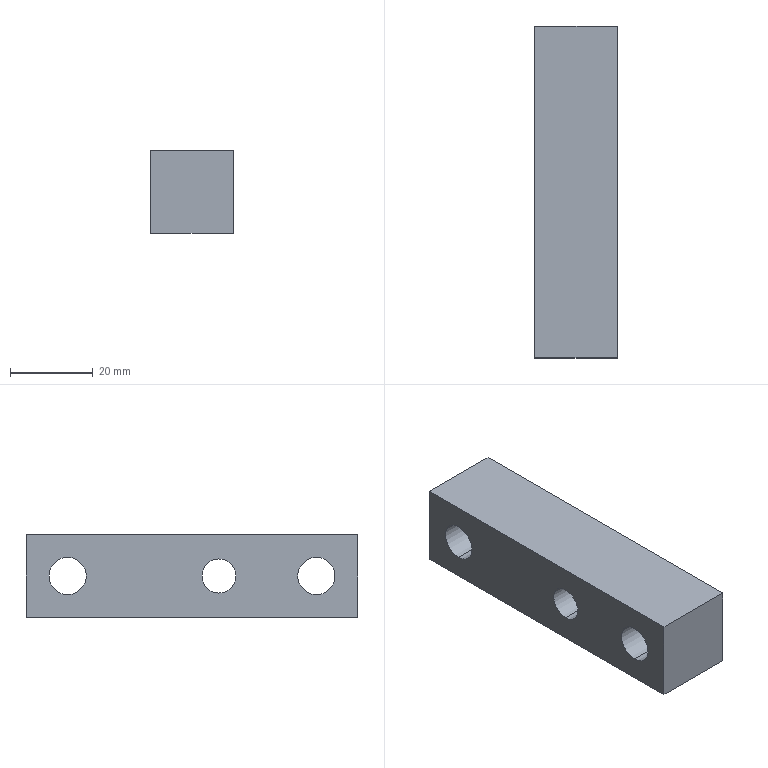Component | SolidWorks | TensionAdjustmentBlock-1 | 1 solid | 18 faces | box 20 x 80 x 20 mm | volume 26954 mm3 | cylinder 10 | plane 8 | commonest cylinder face diameters 14 x4 9 x4 8.2 x2
STEP:
#1=CARTESIAN_POINT('',(11.437,-1.571,25.004));
#2=VERTEX_POINT('',#1);
#3=CARTESIAN_POINT('',(11.437,-1.571,24.681));
#4=VERTEX_POINT('',#3);
#5=CARTESIAN_POINT('',(11.437,-1.571,24.843));
#6=DIRECTION('',(1.,0.,0.));
#7=DIRECTION('',(0.,-0.,-1.));
#8=AXIS2_PLACEMENT_3D('',#5,#6,#7);
#9=CIRCLE('',#8,0.1614);
#10=EDGE_CURVE('',#2,#4,#9,.T.);
#11=ORIENTED_EDGE('',*,*,#10,.F.);
#12=CARTESIAN_POINT('',(12.224,-1.571,25.004));
#13=VERTEX_POINT('',#12);
#14=CARTESIAN_POINT('',(11.437,-1.571,25.004));
#15=DIRECTION('',(1.,0.,0.));
#16=VECTOR('',#15,39.37);
#17=LINE('',#14,#16);
#18=EDGE_CURVE('',#2,#13,#17,.T.);
#19=ORIENTED_EDGE('',*,*,#18,.T.);
#20=CARTESIAN_POINT('',(12.224,-1.571,24.681));
#21=VERTEX_POINT('',#20);
#22=CARTESIAN_POINT('',(12.224,-1.571,24.843));
#23=DIRECTION('',(1.,0.,0.));
#24=DIRECTION('',(0.,-0.,-1.));
#25=AXIS2_PLACEMENT_3D('',#22,#23,#24);
#26=CIRCLE('',#25,0.1614);
#27=EDGE_CURVE('',#13,#21,#26,.T.);
#28=ORIENTED_EDGE('',*,*,#27,.T.);
#29=CARTESIAN_POINT('',(11.437,-1.571,24.681));
#30=DIRECTION('',(1.,0.,0.));
#31=VECTOR('',#30,39.37);
#32=LINE('',#29,#31);
#33=EDGE_CURVE('',#4,#21,#32,.T.);
#34=ORIENTED_EDGE('',*,*,#33,.F.);
#35=EDGE_LOOP('',(#11,#19,#28,#34));
#36=FACE_OUTER_BOUND('',#35,.T.);
#37=CARTESIAN_POINT('',(11.437,-1.571,24.843));
#38=DIRECTION('',(1.,0.,0.));
#39=DIRECTION('',(0.,-0.,-1.));
#40=AXIS2_PLACEMENT_3D('',#37,#38,#39);
#41=CYLINDRICAL_SURFACE('',#40,0.1614);
#42=ADVANCED_FACE('',(#36),#41,.F.);
#43=CARTESIAN_POINT('',(11.909,-0.1343,25.118));
#44=VERTEX_POINT('',#43);
#45=CARTESIAN_POINT('',(11.909,-0.1343,24.567));
#46=VERTEX_POINT('',#45);
#47=CARTESIAN_POINT('',(11.909,-0.1343,24.843));
#48=DIRECTION('',(1.,0.,0.));
#49=DIRECTION('',(0.,-0.,-1.));
#50=AXIS2_PLACEMENT_3D('',#47,#48,#49);
#51=CIRCLE('',#50,0.2756);
#52=EDGE_CURVE('',#44,#46,#51,.T.);
#53=ORIENTED_EDGE('',*,*,#52,.F.);
#54=CARTESIAN_POINT('',(12.224,-0.1343,25.118));
#55=VERTEX_POINT('',#54);
#56=CARTESIAN_POINT('',(12.224,-0.1343,25.118));
#57=DIRECTION('',(1.,0.,0.));
#58=VECTOR('',#57,39.37);
#59=LINE('',#56,#58);
#60=EDGE_CURVE('',#44,#55,#59,.T.);
#61=ORIENTED_EDGE('',*,*,#60,.T.);
#62=CARTESIAN_POINT('',(12.224,-0.1343,24.567));
#63=VERTEX_POINT('',#62);
#64=CARTESIAN_POINT('',(12.224,-0.1343,24.843));
#65=DIRECTION('',(1.,0.,0.));
#66=DIRECTION('',(0.,-0.,-1.));
#67=AXIS2_PLACEMENT_3D('',#64,#65,#66);
#68=CIRCLE('',#67,0.2756);
#69=EDGE_CURVE('',#55,#63,#68,.T.);
#70=ORIENTED_EDGE('',*,*,#69,.T.);
#71=CARTESIAN_POINT('',(12.224,-0.1343,24.567));
#72=DIRECTION('',(1.,0.,0.));
#73=VECTOR('',#72,39.37);
#74=LINE('',#71,#73);
#75=EDGE_CURVE('',#46,#63,#74,.T.);
#76=ORIENTED_EDGE('',*,*,#75,.F.);
#77=EDGE_LOOP('',(#53,#61,#70,#76));
#78=FACE_OUTER_BOUND('',#77,.T.);
#79=CARTESIAN_POINT('',(12.224,-0.1343,24.843));
#80=DIRECTION('',(1.,0.,0.));
#81=DIRECTION('',(0.,-0.,-1.));
#82=AXIS2_PLACEMENT_3D('',#79,#80,#81);
#83=CYLINDRICAL_SURFACE('',#82,0.2756);
#84=ADVANCED_FACE('',(#78),#83,.F.);
#85=CARTESIAN_POINT('',(11.437,-0.1343,25.02));
#86=VERTEX_POINT('',#85);
#87=CARTESIAN_POINT('',(11.437,-0.1343,24.665));
#88=VERTEX_POINT('',#87);
#89=CARTESIAN_POINT('',(11.437,-0.1343,24.843));
#90=DIRECTION('',(1.,0.,0.));
#91=DIRECTION('',(0.,-0.,-1.));
#92=AXIS2_PLACEMENT_3D('',#89,#90,#91);
#93=CIRCLE('',#92,0.1772);
#94=EDGE_CURVE('',#86,#88,#93,.T.);
#95=ORIENTED_EDGE('',*,*,#94,.F.);
#96=CARTESIAN_POINT('',(11.909,-0.1343,25.02));
#97=VERTEX_POINT('',#96);
#98=CARTESIAN_POINT('',(12.224,-0.1343,25.02));
#99=DIRECTION('',(1.,0.,0.));
#100=VECTOR('',#99,39.37);
#101=LINE('',#98,#100);
#102=EDGE_CURVE('',#86,#97,#101,.T.);
#103=ORIENTED_EDGE('',*,*,#102,.T.);
#104=CARTESIAN_POINT('',(11.909,-0.1343,24.665));
#105=VERTEX_POINT('',#104);
#106=CARTESIAN_POINT('',(11.909,-0.1343,24.843));
#107=DIRECTION('',(1.,0.,0.));
#108=DIRECTION('',(0.,-0.,-1.));
#109=AXIS2_PLACEMENT_3D('',#106,#107,#108);
#110=CIRCLE('',#109,0.1772);
#111=EDGE_CURVE('',#97,#105,#110,.T.);
#112=ORIENTED_EDGE('',*,*,#111,.T.);
#113=CARTESIAN_POINT('',(12.224,-0.1343,24.665));
#114=DIRECTION('',(1.,0.,0.));
#115=VECTOR('',#114,39.37);
#116=LINE('',#113,#115);
#117=EDGE_CURVE('',#88,#105,#116,.T.);
#118=ORIENTED_EDGE('',*,*,#117,.F.);
#119=EDGE_LOOP('',(#95,#103,#112,#118));
#120=FACE_OUTER_BOUND('',#119,.T.);
#121=CARTESIAN_POINT('',(12.224,-0.1343,24.843));
#122=DIRECTION('',(1.,0.,0.));
#123=DIRECTION('',(0.,-0.,-1.));
#124=AXIS2_PLACEMENT_3D('',#121,#122,#123);
#125=CYLINDRICAL_SURFACE('',#124,0.1772);
#126=ADVANCED_FACE('',(#120),#125,.F.);
#127=CARTESIAN_POINT('',(11.909,-2.497,25.118));
#128=VERTEX_POINT('',#127);
#129=CARTESIAN_POINT('',(11.909,-2.497,24.567));
#130=VERTEX_POINT('',#129);
#131=CARTESIAN_POINT('',(11.909,-2.497,24.843));
#132=DIRECTION('',(1.,0.,0.));
#133=DIRECTION('',(0.,-0.,-1.));
#134=AXIS2_PLACEMENT_3D('',#131,#132,#133);
#135=CIRCLE('',#134,0.2756);
#136=EDGE_CURVE('',#128,#130,#135,.T.);
#137=ORIENTED_EDGE('',*,*,#136,.F.);
#138=CARTESIAN_POINT('',(12.224,-2.497,25.118));
#139=VERTEX_POINT('',#138);
#140=CARTESIAN_POINT('',(12.224,-2.497,25.118));
#141=DIRECTION('',(1.,0.,0.));
#142=VECTOR('',#141,39.37);
#143=LINE('',#140,#142);
#144=EDGE_CURVE('',#128,#139,#143,.T.);
#145=ORIENTED_EDGE('',*,*,#144,.T.);
#146=CARTESIAN_POINT('',(12.224,-2.497,24.567));
#147=VERTEX_POINT('',#146);
#148=CARTESIAN_POINT('',(12.224,-2.497,24.843));
#149=DIRECTION('',(1.,0.,0.));
#150=DIRECTION('',(0.,-0.,-1.));
#151=AXIS2_PLACEMENT_3D('',#148,#149,#150);
#152=CIRCLE('',#151,0.2756);
#153=EDGE_CURVE('',#139,#147,#152,.T.);
#154=ORIENTED_EDGE('',*,*,#153,.T.);
#155=CARTESIAN_POINT('',(12.224,-2.497,24.567));
#156=DIRECTION('',(1.,0.,0.));
#157=VECTOR('',#156,39.37);
#158=LINE('',#155,#157);
#159=EDGE_CURVE('',#130,#147,#158,.T.);
#160=ORIENTED_EDGE('',*,*,#159,.F.);
#161=EDGE_LOOP('',(#137,#145,#154,#160));
#162=FACE_OUTER_BOUND('',#161,.T.);
#163=CARTESIAN_POINT('',(12.224,-2.497,24.843));
#164=DIRECTION('',(1.,0.,0.));
#165=DIRECTION('',(0.,-0.,-1.));
#166=AXIS2_PLACEMENT_3D('',#163,#164,#165);
#167=CYLINDRICAL_SURFACE('',#166,0.2756);
#168=ADVANCED_FACE('',(#162),#167,.F.);
#169=CARTESIAN_POINT('',(11.437,-2.497,25.02));
#170=VERTEX_POINT('',#169);
#171=CARTESIAN_POINT('',(11.437,-2.497,24.665));
#172=VERTEX_POINT('',#171);
#173=CARTESIAN_POINT('',(11.437,-2.497,24.843));
#174=DIRECTION('',(1.,0.,0.));
#175=DIRECTION('',(0.,-0.,-1.));
#176=AXIS2_PLACEMENT_3D('',#173,#174,#175);
#177=CIRCLE('',#176,0.1772);
#178=EDGE_CURVE('',#170,#172,#177,.T.);
#179=ORIENTED_EDGE('',*,*,#178,.F.);
#180=CARTESIAN_POINT('',(11.909,-2.497,25.02));
#181=VERTEX_POINT('',#180);
#182=CARTESIAN_POINT('',(12.224,-2.497,25.02));
#183=DIRECTION('',(1.,0.,0.));
#184=VECTOR('',#183,39.37);
#185=LINE('',#182,#184);
#186=EDGE_CURVE('',#170,#181,#185,.T.);
#187=ORIENTED_EDGE('',*,*,#186,.T.);
#188=CARTESIAN_POINT('',(11.909,-2.497,24.665));
#189=VERTEX_POINT('',#188);
#190=CARTESIAN_POINT('',(11.909,-2.497,24.843));
#191=DIRECTION('',(1.,0.,0.));
#192=DIRECTION('',(0.,-0.,-1.));
#193=AXIS2_PLACEMENT_3D('',#190,#191,#192);
#194=CIRCLE('',#193,0.1772);
#195=EDGE_CURVE('',#181,#189,#194,.T.);
#196=ORIENTED_EDGE('',*,*,#195,.T.);
#197=CARTESIAN_POINT('',(12.224,-2.497,24.665));
#198=DIRECTION('',(1.,0.,0.));
#199=VECTOR('',#198,39.37);
#200=LINE('',#197,#199);
#201=EDGE_CURVE('',#172,#189,#200,.T.);
#202=ORIENTED_EDGE('',*,*,#201,.F.);
#203=EDGE_LOOP('',(#179,#187,#196,#202));
#204=FACE_OUTER_BOUND('',#203,.T.);
#205=CARTESIAN_POINT('',(12.224,-2.497,24.843));
#206=DIRECTION('',(1.,0.,0.));
#207=DIRECTION('',(0.,-0.,-1.));
#208=AXIS2_PLACEMENT_3D('',#205,#206,#207);
#209=CYLINDRICAL_SURFACE('',#208,0.1772);
#210=ADVANCED_FACE('',(#204),#209,.F.);
#211=CARTESIAN_POINT('',(11.437,-2.89,24.449));
#212=VERTEX_POINT('',#211);
#213=CARTESIAN_POINT('',(11.437,0.2594,24.449));
#214=VERTEX_POINT('',#213);
#215=CARTESIAN_POINT('',(11.437,0.2594,24.449));
#216=DIRECTION('',(-0.,1.,-0.));
#217=VECTOR('',#216,39.37);
#218=LINE('',#215,#217);
#219=EDGE_CURVE('',#212,#214,#218,.T.);
#220=ORIENTED_EDGE('',*,*,#219,.T.);
#221=CARTESIAN_POINT('',(12.224,0.2594,24.449));
#222=VERTEX_POINT('',#221);
#223=CARTESIAN_POINT('',(12.224,0.2594,24.449));
#224=DIRECTION('',(-1.,-0.,-0.));
#225=VECTOR('',#224,39.37);
#226=LINE('',#223,#225);
#227=EDGE_CURVE('',#222,#214,#226,.T.);
#228=ORIENTED_EDGE('',*,*,#227,.F.);
#229=CARTESIAN_POINT('',(12.224,-2.89,24.449));
#230=VERTEX_POINT('',#229);
#231=CARTESIAN_POINT('',(12.224,0.2594,24.449));
#232=DIRECTION('',(-0.,1.,-0.));
#233=VECTOR('',#232,39.37);
#234=LINE('',#231,#233);
#235=EDGE_CURVE('',#230,#222,#234,.T.);
#236=ORIENTED_EDGE('',*,*,#235,.F.);
#237=CARTESIAN_POINT('',(12.224,-2.89,24.449));
#238=DIRECTION('',(-1.,-0.,-0.));
#239=VECTOR('',#238,39.37);
#240=LINE('',#237,#239);
#241=EDGE_CURVE('',#230,#212,#240,.T.);
#242=ORIENTED_EDGE('',*,*,#241,.T.);
#243=EDGE_LOOP('',(#220,#228,#236,#242));
#244=FACE_OUTER_BOUND('',#243,.T.);
#245=CARTESIAN_POINT('',(12.224,0.2594,24.449));
#246=DIRECTION('',(-0.,0.,1.));
#247=DIRECTION('',(0.,-1.,0.));
#248=AXIS2_PLACEMENT_3D('',#245,#246,#247);
#249=PLANE('',#248);
#250=ADVANCED_FACE('',(#244),#249,.F.);
#251=CARTESIAN_POINT('',(11.437,0.2594,25.236));
#252=VERTEX_POINT('',#251);
#253=CARTESIAN_POINT('',(11.437,0.2594,25.236));
#254=DIRECTION('',(-0.,0.,1.));
#255=VECTOR('',#254,39.37);
#256=LINE('',#253,#255);
#257=EDGE_CURVE('',#214,#252,#256,.T.);
#258=ORIENTED_EDGE('',*,*,#257,.T.);
#259=CARTESIAN_POINT('',(12.224,0.2594,25.236));
#260=VERTEX_POINT('',#259);
#261=CARTESIAN_POINT('',(12.224,0.2594,25.236));
#262=DIRECTION('',(-1.,-0.,-0.));
#263=VECTOR('',#262,39.37);
#264=LINE('',#261,#263);
#265=EDGE_CURVE('',#260,#252,#264,.T.);
#266=ORIENTED_EDGE('',*,*,#265,.F.);
#267=CARTESIAN_POINT('',(12.224,0.2594,25.236));
#268=DIRECTION('',(-0.,0.,1.));
#269=VECTOR('',#268,39.37);
#270=LINE('',#267,#269);
#271=EDGE_CURVE('',#222,#260,#270,.T.);
#272=ORIENTED_EDGE('',*,*,#271,.F.);
#273=ORIENTED_EDGE('',*,*,#227,.T.);
#274=EDGE_LOOP('',(#258,#266,#272,#273));
#275=FACE_OUTER_BOUND('',#274,.T.);
#276=CARTESIAN_POINT('',(12.224,0.2594,25.236));
#277=DIRECTION('',(0.,-1.,0.));
#278=DIRECTION('',(-1.,-0.,-0.));
#279=AXIS2_PLACEMENT_3D('',#276,#277,#278);
#280=PLANE('',#279);
#281=ADVANCED_FACE('',(#275),#280,.F.);
#282=CARTESIAN_POINT('',(11.437,-2.89,25.236));
#283=VERTEX_POINT('',#282);
#284=CARTESIAN_POINT('',(11.437,0.2594,25.236));
#285=DIRECTION('',(0.,-1.,0.));
#286=VECTOR('',#285,39.37);
#287=LINE('',#284,#286);
#288=EDGE_CURVE('',#252,#283,#287,.T.);
#289=ORIENTED_EDGE('',*,*,#288,.T.);
#290=CARTESIAN_POINT('',(12.224,-2.89,25.236));
#291=VERTEX_POINT('',#290);
#292=CARTESIAN_POINT('',(12.224,-2.89,25.236));
#293=DIRECTION('',(-1.,-0.,-0.));
#294=VECTOR('',#293,39.37);
#295=LINE('',#292,#294);
#296=EDGE_CURVE('',#291,#283,#295,.T.);
#297=ORIENTED_EDGE('',*,*,#296,.F.);
#298=CARTESIAN_POINT('',(12.224,0.2594,25.236));
#299=DIRECTION('',(0.,-1.,0.));
#300=VECTOR('',#299,39.37);
#301=LINE('',#298,#300);
#302=EDGE_CURVE('',#260,#291,#301,.T.);
#303=ORIENTED_EDGE('',*,*,#302,.F.);
#304=ORIENTED_EDGE('',*,*,#265,.T.);
#305=EDGE_LOOP('',(#289,#297,#303,#304));
#306=FACE_OUTER_BOUND('',#305,.T.);
#307=CARTESIAN_POINT('',(12.224,0.2594,25.236));
#308=DIRECTION('',(0.,-0.,-1.));
#309=DIRECTION('',(-0.,1.,-0.));
#310=AXIS2_PLACEMENT_3D('',#307,#308,#309);
#311=PLANE('',#310);
#312=ADVANCED_FACE('',(#306),#311,.F.);
#313=CARTESIAN_POINT('',(11.437,-2.89,25.236));
#314=DIRECTION('',(0.,-0.,-1.));
#315=VECTOR('',#314,39.37);
#316=LINE('',#313,#315);
#317=EDGE_CURVE('',#283,#212,#316,.T.);
#318=ORIENTED_EDGE('',*,*,#317,.T.);
#319=ORIENTED_EDGE('',*,*,#241,.F.);
#320=CARTESIAN_POINT('',(12.224,-2.89,25.236));
#321=DIRECTION('',(0.,-0.,-1.));
#322=VECTOR('',#321,39.37);
#323=LINE('',#320,#322);
#324=EDGE_CURVE('',#291,#230,#323,.T.);
#325=ORIENTED_EDGE('',*,*,#324,.F.);
#326=ORIENTED_EDGE('',*,*,#296,.T.);
#327=EDGE_LOOP('',(#318,#319,#325,#326));
#328=FACE_OUTER_BOUND('',#327,.T.);
#329=CARTESIAN_POINT('',(12.224,-2.89,25.236));
#330=DIRECTION('',(-0.,1.,-0.));
#331=DIRECTION('',(1.,0.,0.));
#332=AXIS2_PLACEMENT_3D('',#329,#330,#331);
#333=PLANE('',#332);
#334=ADVANCED_FACE('',(#328),#333,.F.);
#335=CARTESIAN_POINT('',(12.224,-1.571,24.843));
#336=DIRECTION('',(1.,0.,0.));
#337=DIRECTION('',(0.,-0.,-1.));
#338=AXIS2_PLACEMENT_3D('',#335,#336,#337);
#339=CIRCLE('',#338,0.1614);
#340=EDGE_CURVE('',#21,#13,#339,.T.);
#341=ORIENTED_EDGE('',*,*,#340,.F.);
#342=ORIENTED_EDGE('',*,*,#27,.F.);
#343=EDGE_LOOP('',(#341,#342));
#344=FACE_BOUND('',#343,.T.);
#345=CARTESIAN_POINT('',(12.224,-0.1343,24.843));
#346=DIRECTION('',(1.,0.,0.));
#347=DIRECTION('',(0.,-0.,-1.));
#348=AXIS2_PLACEMENT_3D('',#345,#346,#347);
#349=CIRCLE('',#348,0.2756);
#350=EDGE_CURVE('',#63,#55,#349,.T.);
#351=ORIENTED_EDGE('',*,*,#350,.F.);
#352=ORIENTED_EDGE('',*,*,#69,.F.);
#353=EDGE_LOOP('',(#351,#352));
#354=FACE_BOUND('',#353,.T.);
#355=CARTESIAN_POINT('',(12.224,-2.497,24.843));
#356=DIRECTION('',(1.,0.,0.));
#357=DIRECTION('',(0.,-0.,-1.));
#358=AXIS2_PLACEMENT_3D('',#355,#356,#357);
#359=CIRCLE('',#358,0.2756);
#360=EDGE_CURVE('',#147,#139,#359,.T.);
#361=ORIENTED_EDGE('',*,*,#360,.F.);
#362=ORIENTED_EDGE('',*,*,#153,.F.);
#363=EDGE_LOOP('',(#361,#362));
#364=FACE_BOUND('',#363,.T.);
#365=ORIENTED_EDGE('',*,*,#235,.T.);
#366=ORIENTED_EDGE('',*,*,#271,.T.);
#367=ORIENTED_EDGE('',*,*,#302,.T.);
#368=ORIENTED_EDGE('',*,*,#324,.T.);
#369=EDGE_LOOP('',(#365,#366,#367,#368));
#370=FACE_OUTER_BOUND('',#369,.T.);
#371=CARTESIAN_POINT('',(12.224,-1.315,24.843));
#372=DIRECTION('',(1.,0.,0.));
#373=DIRECTION('',(0.,-0.,-1.));
#374=AXIS2_PLACEMENT_3D('',#371,#372,#373);
#375=PLANE('',#374);
#376=ADVANCED_FACE('',(#344,#354,#364,#370),#375,.T.);
#377=CARTESIAN_POINT('',(11.437,-1.571,24.843));
#378=DIRECTION('',(1.,0.,0.));
#379=DIRECTION('',(0.,-0.,-1.));
#380=AXIS2_PLACEMENT_3D('',#377,#378,#379);
#381=CIRCLE('',#380,0.1614);
#382=EDGE_CURVE('',#4,#2,#381,.T.);
#383=ORIENTED_EDGE('',*,*,#382,.T.);
#384=ORIENTED_EDGE('',*,*,#10,.T.);
#385=EDGE_LOOP('',(#383,#384));
#386=FACE_BOUND('',#385,.T.);
#387=CARTESIAN_POINT('',(11.437,-0.1343,24.843));
#388=DIRECTION('',(1.,0.,0.));
#389=DIRECTION('',(0.,-0.,-1.));
#390=AXIS2_PLACEMENT_3D('',#387,#388,#389);
#391=CIRCLE('',#390,0.1772);
#392=EDGE_CURVE('',#88,#86,#391,.T.);
#393=ORIENTED_EDGE('',*,*,#392,.T.);
#394=ORIENTED_EDGE('',*,*,#94,.T.);
#395=EDGE_LOOP('',(#393,#394));
#396=FACE_BOUND('',#395,.T.);
#397=CARTESIAN_POINT('',(11.437,-2.497,24.843));
#398=DIRECTION('',(1.,0.,0.));
#399=DIRECTION('',(0.,-0.,-1.));
#400=AXIS2_PLACEMENT_3D('',#397,#398,#399);
#401=CIRCLE('',#400,0.1772);
#402=EDGE_CURVE('',#172,#170,#401,.T.);
#403=ORIENTED_EDGE('',*,*,#402,.T.);
#404=ORIENTED_EDGE('',*,*,#178,.T.);
#405=EDGE_LOOP('',(#403,#404));
#406=FACE_BOUND('',#405,.T.);
#407=ORIENTED_EDGE('',*,*,#219,.F.);
#408=ORIENTED_EDGE('',*,*,#317,.F.);
#409=ORIENTED_EDGE('',*,*,#288,.F.);
#410=ORIENTED_EDGE('',*,*,#257,.F.);
#411=EDGE_LOOP('',(#407,#408,#409,#410));
#412=FACE_OUTER_BOUND('',#411,.T.);
#413=CARTESIAN_POINT('',(11.437,-1.315,24.843));
#414=DIRECTION('',(1.,0.,0.));
#415=DIRECTION('',(0.,-0.,-1.));
#416=AXIS2_PLACEMENT_3D('',#413,#414,#415);
#417=PLANE('',#416);
#418=ADVANCED_FACE('',(#386,#396,#406,#412),#417,.F.);
#419=ORIENTED_EDGE('',*,*,#186,.F.);
#420=ORIENTED_EDGE('',*,*,#402,.F.);
#421=ORIENTED_EDGE('',*,*,#201,.T.);
#422=CARTESIAN_POINT('',(11.909,-2.497,24.843));
#423=DIRECTION('',(1.,0.,0.));
#424=DIRECTION('',(0.,-0.,-1.));
#425=AXIS2_PLACEMENT_3D('',#422,#423,#424);
#426=CIRCLE('',#425,0.1772);
#427=EDGE_CURVE('',#189,#181,#426,.T.);
#428=ORIENTED_EDGE('',*,*,#427,.T.);
#429=EDGE_LOOP('',(#419,#420,#421,#428));
#430=FACE_OUTER_BOUND('',#429,.T.);
#431=CARTESIAN_POINT('',(12.224,-2.497,24.843));
#432=DIRECTION('',(1.,0.,0.));
#433=DIRECTION('',(0.,-0.,-1.));
#434=AXIS2_PLACEMENT_3D('',#431,#432,#433);
#435=CYLINDRICAL_SURFACE('',#434,0.1772);
#436=ADVANCED_FACE('',(#430),#435,.F.);
#437=ORIENTED_EDGE('',*,*,#427,.F.);
#438=ORIENTED_EDGE('',*,*,#195,.F.);
#439=EDGE_LOOP('',(#437,#438));
#440=FACE_BOUND('',#439,.T.);
#441=CARTESIAN_POINT('',(11.909,-2.497,24.843));
#442=DIRECTION('',(1.,0.,0.));
#443=DIRECTION('',(0.,-0.,-1.));
#444=AXIS2_PLACEMENT_3D('',#441,#442,#443);
#445=CIRCLE('',#444,0.2756);
#446=EDGE_CURVE('',#130,#128,#445,.T.);
#447=ORIENTED_EDGE('',*,*,#446,.T.);
#448=ORIENTED_EDGE('',*,*,#136,.T.);
#449=EDGE_LOOP('',(#447,#448));
#450=FACE_OUTER_BOUND('',#449,.T.);
#451=CARTESIAN_POINT('',(11.909,-2.497,24.665));
#452=DIRECTION('',(-1.,-0.,-0.));
#453=DIRECTION('',(-0.,0.,1.));
#454=AXIS2_PLACEMENT_3D('',#451,#452,#453);
#455=PLANE('',#454);
#456=ADVANCED_FACE('',(#440,#450),#455,.F.);
#457=ORIENTED_EDGE('',*,*,#144,.F.);
#458=ORIENTED_EDGE('',*,*,#446,.F.);
#459=ORIENTED_EDGE('',*,*,#159,.T.);
#460=ORIENTED_EDGE('',*,*,#360,.T.);
#461=EDGE_LOOP('',(#457,#458,#459,#460));
#462=FACE_OUTER_BOUND('',#461,.T.);
#463=CARTESIAN_POINT('',(12.224,-2.497,24.843));
#464=DIRECTION('',(1.,0.,0.));
#465=DIRECTION('',(0.,-0.,-1.));
#466=AXIS2_PLACEMENT_3D('',#463,#464,#465);
#467=CYLINDRICAL_SURFACE('',#466,0.2756);
#468=ADVANCED_FACE('',(#462),#467,.F.);
#469=ORIENTED_EDGE('',*,*,#102,.F.);
#470=ORIENTED_EDGE('',*,*,#392,.F.);
#471=ORIENTED_EDGE('',*,*,#117,.T.);
#472=CARTESIAN_POINT('',(11.909,-0.1343,24.843));
#473=DIRECTION('',(1.,0.,0.));
#474=DIRECTION('',(0.,-0.,-1.));
#475=AXIS2_PLACEMENT_3D('',#472,#473,#474);
#476=CIRCLE('',#475,0.1772);
#477=EDGE_CURVE('',#105,#97,#476,.T.);
#478=ORIENTED_EDGE('',*,*,#477,.T.);
#479=EDGE_LOOP('',(#469,#470,#471,#478));
#480=FACE_OUTER_BOUND('',#479,.T.);
#481=CARTESIAN_POINT('',(12.224,-0.1343,24.843));
#482=DIRECTION('',(1.,0.,0.));
#483=DIRECTION('',(0.,-0.,-1.));
#484=AXIS2_PLACEMENT_3D('',#481,#482,#483);
#485=CYLINDRICAL_SURFACE('',#484,0.1772);
#486=ADVANCED_FACE('',(#480),#485,.F.);
#487=ORIENTED_EDGE('',*,*,#477,.F.);
#488=ORIENTED_EDGE('',*,*,#111,.F.);
#489=EDGE_LOOP('',(#487,#488));
#490=FACE_BOUND('',#489,.T.);
#491=CARTESIAN_POINT('',(11.909,-0.1343,24.843));
#492=DIRECTION('',(1.,0.,0.));
#493=DIRECTION('',(0.,-0.,-1.));
#494=AXIS2_PLACEMENT_3D('',#491,#492,#493);
#495=CIRCLE('',#494,0.2756);
#496=EDGE_CURVE('',#46,#44,#495,.T.);
#497=ORIENTED_EDGE('',*,*,#496,.T.);
#498=ORIENTED_EDGE('',*,*,#52,.T.);
#499=EDGE_LOOP('',(#497,#498));
#500=FACE_OUTER_BOUND('',#499,.T.);
#501=CARTESIAN_POINT('',(11.909,-0.1343,24.665));
#502=DIRECTION('',(-1.,-0.,-0.));
#503=DIRECTION('',(-0.,0.,1.));
#504=AXIS2_PLACEMENT_3D('',#501,#502,#503);
#505=PLANE('',#504);
#506=ADVANCED_FACE('',(#490,#500),#505,.F.);
#507=ORIENTED_EDGE('',*,*,#60,.F.);
#508=ORIENTED_EDGE('',*,*,#496,.F.);
#509=ORIENTED_EDGE('',*,*,#75,.T.);
#510=ORIENTED_EDGE('',*,*,#350,.T.);
#511=EDGE_LOOP('',(#507,#508,#509,#510));
#512=FACE_OUTER_BOUND('',#511,.T.);
#513=CARTESIAN_POINT('',(12.224,-0.1343,24.843));
#514=DIRECTION('',(1.,0.,0.));
#515=DIRECTION('',(0.,-0.,-1.));
#516=AXIS2_PLACEMENT_3D('',#513,#514,#515);
#517=CYLINDRICAL_SURFACE('',#516,0.2756);
#518=ADVANCED_FACE('',(#512),#517,.F.);
#519=ORIENTED_EDGE('',*,*,#18,.F.);
#520=ORIENTED_EDGE('',*,*,#382,.F.);
#521=ORIENTED_EDGE('',*,*,#33,.T.);
#522=ORIENTED_EDGE('',*,*,#340,.T.);
#523=EDGE_LOOP('',(#519,#520,#521,#522));
#524=FACE_OUTER_BOUND('',#523,.T.);
#525=CARTESIAN_POINT('',(11.437,-1.571,24.843));
#526=DIRECTION('',(1.,0.,0.));
#527=DIRECTION('',(0.,-0.,-1.));
#528=AXIS2_PLACEMENT_3D('',#525,#526,#527);
#529=CYLINDRICAL_SURFACE('',#528,0.1614);
#530=ADVANCED_FACE('',(#524),#529,.F.);
#531=CLOSED_SHELL('',(#42,#84,#126,#168,#210,#250,#281,#312,#334,#376,#418,#436,#456,#468,#486,#506,#518,#530));
#532=MANIFOLD_SOLID_BREP('',#531);
#533=CARTESIAN_POINT('',(0.,0.,0.));
#534=DIRECTION('',(0.,0.,1.));
#535=DIRECTION('',(1.,0.,0.));
#536=AXIS2_PLACEMENT_3D('',#533,#534,#535);
#537=(LENGTH_UNIT()NAMED_UNIT(*)SI_UNIT($,.METRE.));
#538=LENGTH_MEASURE_WITH_UNIT(LENGTH_MEASURE(0.0254),#537);
#539=DIMENSIONAL_EXPONENTS(1.,0.,0.,0.,0.,0.,0.);
#540=(CONVERSION_BASED_UNIT('',#538)LENGTH_UNIT()NAMED_UNIT(#539));
#541=UNCERTAINTY_MEASURE_WITH_UNIT(LENGTH_MEASURE(0.00001),#540,'','');
#542=(NAMED_UNIT(*)PLANE_ANGLE_UNIT()SI_UNIT($,.RADIAN.));
#543=(NAMED_UNIT(*)SI_UNIT($,.STERADIAN.)SOLID_ANGLE_UNIT());
#544=(GEOMETRIC_REPRESENTATION_CONTEXT(3)GLOBAL_UNCERTAINTY_ASSIGNED_CONTEXT((#541))GLOBAL_UNIT_ASSIGNED_CONTEXT((#540,#542,#543))REPRESENTATION_CONTEXT('',''));
#545=ADVANCED_BREP_SHAPE_REPRESENTATION('',(#532,#536),#544);
#546=COLOUR_RGB('',0.7922,0.8196,0.9333);
#547=FILL_AREA_STYLE_COLOUR('',#546);
#548=FILL_AREA_STYLE('',(#547));
#549=SURFACE_STYLE_FILL_AREA(#548);
#550=SURFACE_SIDE_STYLE('',(#549));
#551=SURFACE_STYLE_USAGE(.BOTH.,#550);
#552=PRESENTATION_STYLE_ASSIGNMENT((#551));
#553=STYLED_ITEM('',(#552),#532);
#554=(LENGTH_UNIT()NAMED_UNIT(*)SI_UNIT($,.METRE.));
#555=LENGTH_MEASURE_WITH_UNIT(LENGTH_MEASURE(0.0254),#554);
#556=DIMENSIONAL_EXPONENTS(1.,0.,0.,0.,0.,0.,0.);
#557=(CONVERSION_BASED_UNIT('',#555)LENGTH_UNIT()NAMED_UNIT(#556));
#558=UNCERTAINTY_MEASURE_WITH_UNIT(LENGTH_MEASURE(0.00001),#557,'','');
#559=(NAMED_UNIT(*)PLANE_ANGLE_UNIT()SI_UNIT($,.RADIAN.));
#560=(NAMED_UNIT(*)SI_UNIT($,.STERADIAN.)SOLID_ANGLE_UNIT());
#561=(GEOMETRIC_REPRESENTATION_CONTEXT(3)GLOBAL_UNCERTAINTY_ASSIGNED_CONTEXT((#558))GLOBAL_UNIT_ASSIGNED_CONTEXT((#557,#559,#560))REPRESENTATION_CONTEXT('',''));
#562=MECHANICAL_DESIGN_GEOMETRIC_PRESENTATION_REPRESENTATION('',(#553),#561);
#563=PRESENTATION_LAYER_ASSIGNMENT('','',(#553));